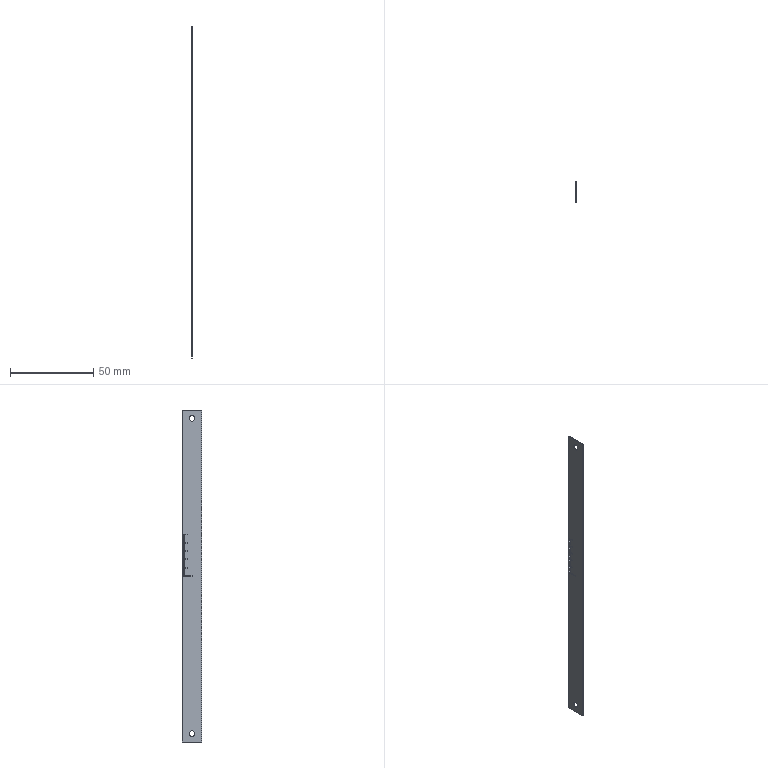Component | SolidWorks | BLR41-L200-1 | 1 solid | 114 faces | box 0.5 x 12 x 200 mm | volume 1185 mm3 | plane 110 | cylinder 4 | commonest cylinder face diameters 3.5 x4
build123d program:
from build123d import *

# Parameters (mm, degrees)
SKETCH1_W           = 0.5
SKETCH1_H           = 12
BOSS_EXTRUDE1_DEPTH = 200
SKETCH2_R           = 1.75
CUT_EXTRUDE1_DEPTH  = 0.5
SKETCH3_R           = 1.75
CUT_EXTRUDE2_DEPTH  = 0.5
SKETCH4_W           = 0.5
SKETCH4_H           = 1.5
SKETCH4_H_2         = 6
SKETCH4_H_3         = 3
CUT_EXTRUDE3_DEPTH  = 0.2


with BuildPart() as part:
    # Sketch1 → Boss-Extrude1 (new body)
    with BuildSketch(Plane(origin=(0, 0, 0), x_dir=(0, 0, -1), z_dir=(1, 0, 0))):
        with Locations((0.25, 6)):
            Rectangle(SKETCH1_W, SKETCH1_H)
    extrude(amount=BOSS_EXTRUDE1_DEPTH)

    # Sketch2 → Cut-Extrude1 (cut)
    with BuildSketch(Plane.XY):
        with Locations((5, 6)):
            Circle(SKETCH2_R)
    extrude(amount=-CUT_EXTRUDE1_DEPTH, mode=Mode.SUBTRACT)

    # Sketch3 → Cut-Extrude2 (cut)
    with BuildSketch(Plane.XY):
        with Locations((195, 6)):
            Circle(SKETCH3_R)
    extrude(amount=-CUT_EXTRUDE2_DEPTH, mode=Mode.SUBTRACT)

    # Sketch4 → Cut-Extrude3 (cut)
    with BuildSketch(Plane(origin=(0, 0, -0.5), x_dir=(-1, 0, 0), z_dir=(0, 0, -1))):
        with Locations((-98, 11.25)):
            Rectangle(SKETCH4_W, SKETCH4_H)
        with Locations((-100, 9)):
            Rectangle(SKETCH4_W, SKETCH4_H_2)
        with Locations((-99, 11.25)):
            Rectangle(SKETCH4_W, SKETCH4_H)
        with Locations((-97, 11.25)):
            Rectangle(SKETCH4_W, SKETCH4_H)
        with Locations((-96, 11.25)):
            Rectangle(SKETCH4_W, SKETCH4_H)
        with Locations((-90, 10.5)):
            Rectangle(SKETCH4_W, SKETCH4_H_3)
        with Locations((-95, 10.5)):
            Rectangle(SKETCH4_W, SKETCH4_H_3)
        with Locations((-91, 11.25)):
            Rectangle(SKETCH4_W, SKETCH4_H)
        with Locations((-92, 11.25)):
            Rectangle(SKETCH4_W, SKETCH4_H)
        with Locations((-93, 11.25)):
            Rectangle(SKETCH4_W, SKETCH4_H)
        with Locations((-94, 11.25)):
            Rectangle(SKETCH4_W, SKETCH4_H)
        with Locations((-85, 10.5)):
            Rectangle(SKETCH4_W, SKETCH4_H_3)
        with Locations((-86, 11.25)):
            Rectangle(SKETCH4_W, SKETCH4_H)
        with Locations((-87, 11.25)):
            Rectangle(SKETCH4_W, SKETCH4_H)
        with Locations((-88, 11.25)):
            Rectangle(SKETCH4_W, SKETCH4_H)
        with Locations((-89, 11.25)):
            Rectangle(SKETCH4_W, SKETCH4_H)
        with Locations((-80, 10.5)):
            Rectangle(SKETCH4_W, SKETCH4_H_3)
        with Locations((-81, 11.25)):
            Rectangle(SKETCH4_W, SKETCH4_H)
        with Locations((-82, 11.25)):
            Rectangle(SKETCH4_W, SKETCH4_H)
        with Locations((-83, 11.25)):
            Rectangle(SKETCH4_W, SKETCH4_H)
        with Locations((-84, 11.25)):
            Rectangle(SKETCH4_W, SKETCH4_H)
        with Locations((-75, 10.5)):
            Rectangle(SKETCH4_W, SKETCH4_H_3)
        with Locations((-76, 11.25)):
            Rectangle(SKETCH4_W, SKETCH4_H)
        with Locations((-77, 11.25)):
            Rectangle(SKETCH4_W, SKETCH4_H)
        with Locations((-78, 11.25)):
            Rectangle(SKETCH4_W, SKETCH4_H)
        with Locations((-79, 11.25)):
            Rectangle(SKETCH4_W, SKETCH4_H)
    extrude(amount=-CUT_EXTRUDE3_DEPTH, mode=Mode.SUBTRACT)


solid = part.part

# Placed as in the assembly
solid = solid.moved(Location((49.798, 45.781, 393.447), (0, 90, 0)))